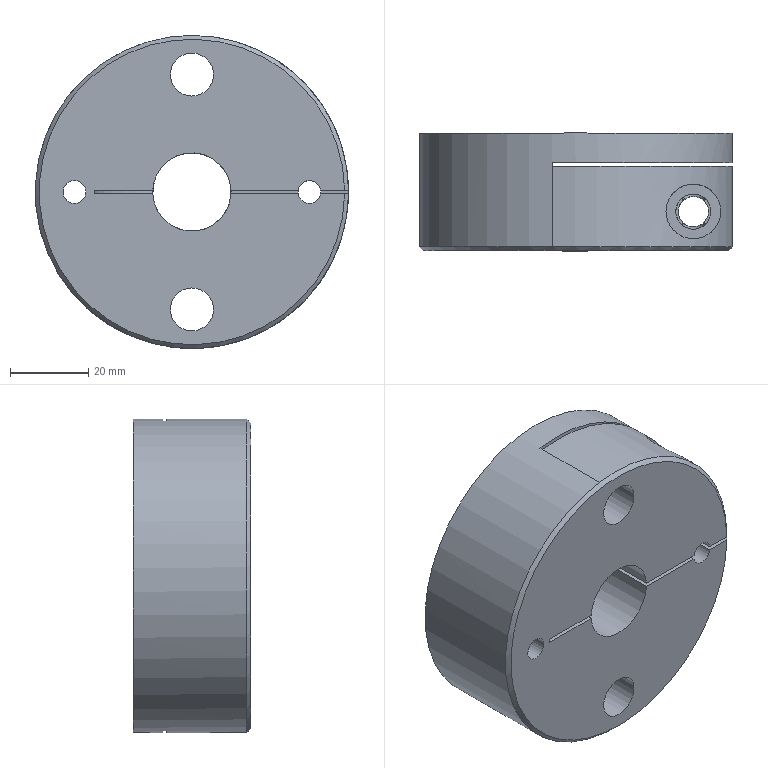Component | NX | HALF_DIAPHRAGM_COUPLING_2 | 1 solid | 33 faces | volume 126619 mm3 | cylinder 18 | plane 14 | cone 1 | commonest cylinder face diameters 5.795 x6 11 x4 80 x2 20 x2 14 x1 50 x1 9 x1 7.76 x1